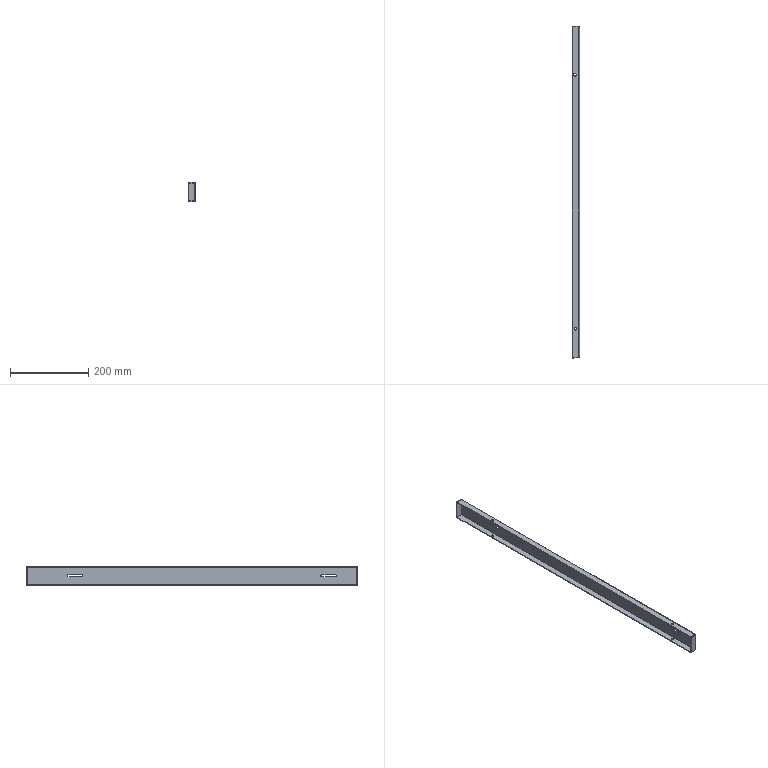Component | SolidWorks | SideFixingBeam-1 | 1 solid | 56 faces | volume 137852 mm3 | plane 26 | cylinder 22 | spline 8 | commonest cylinder face diameters 7 x8 5 x6 6 x4 2 x4